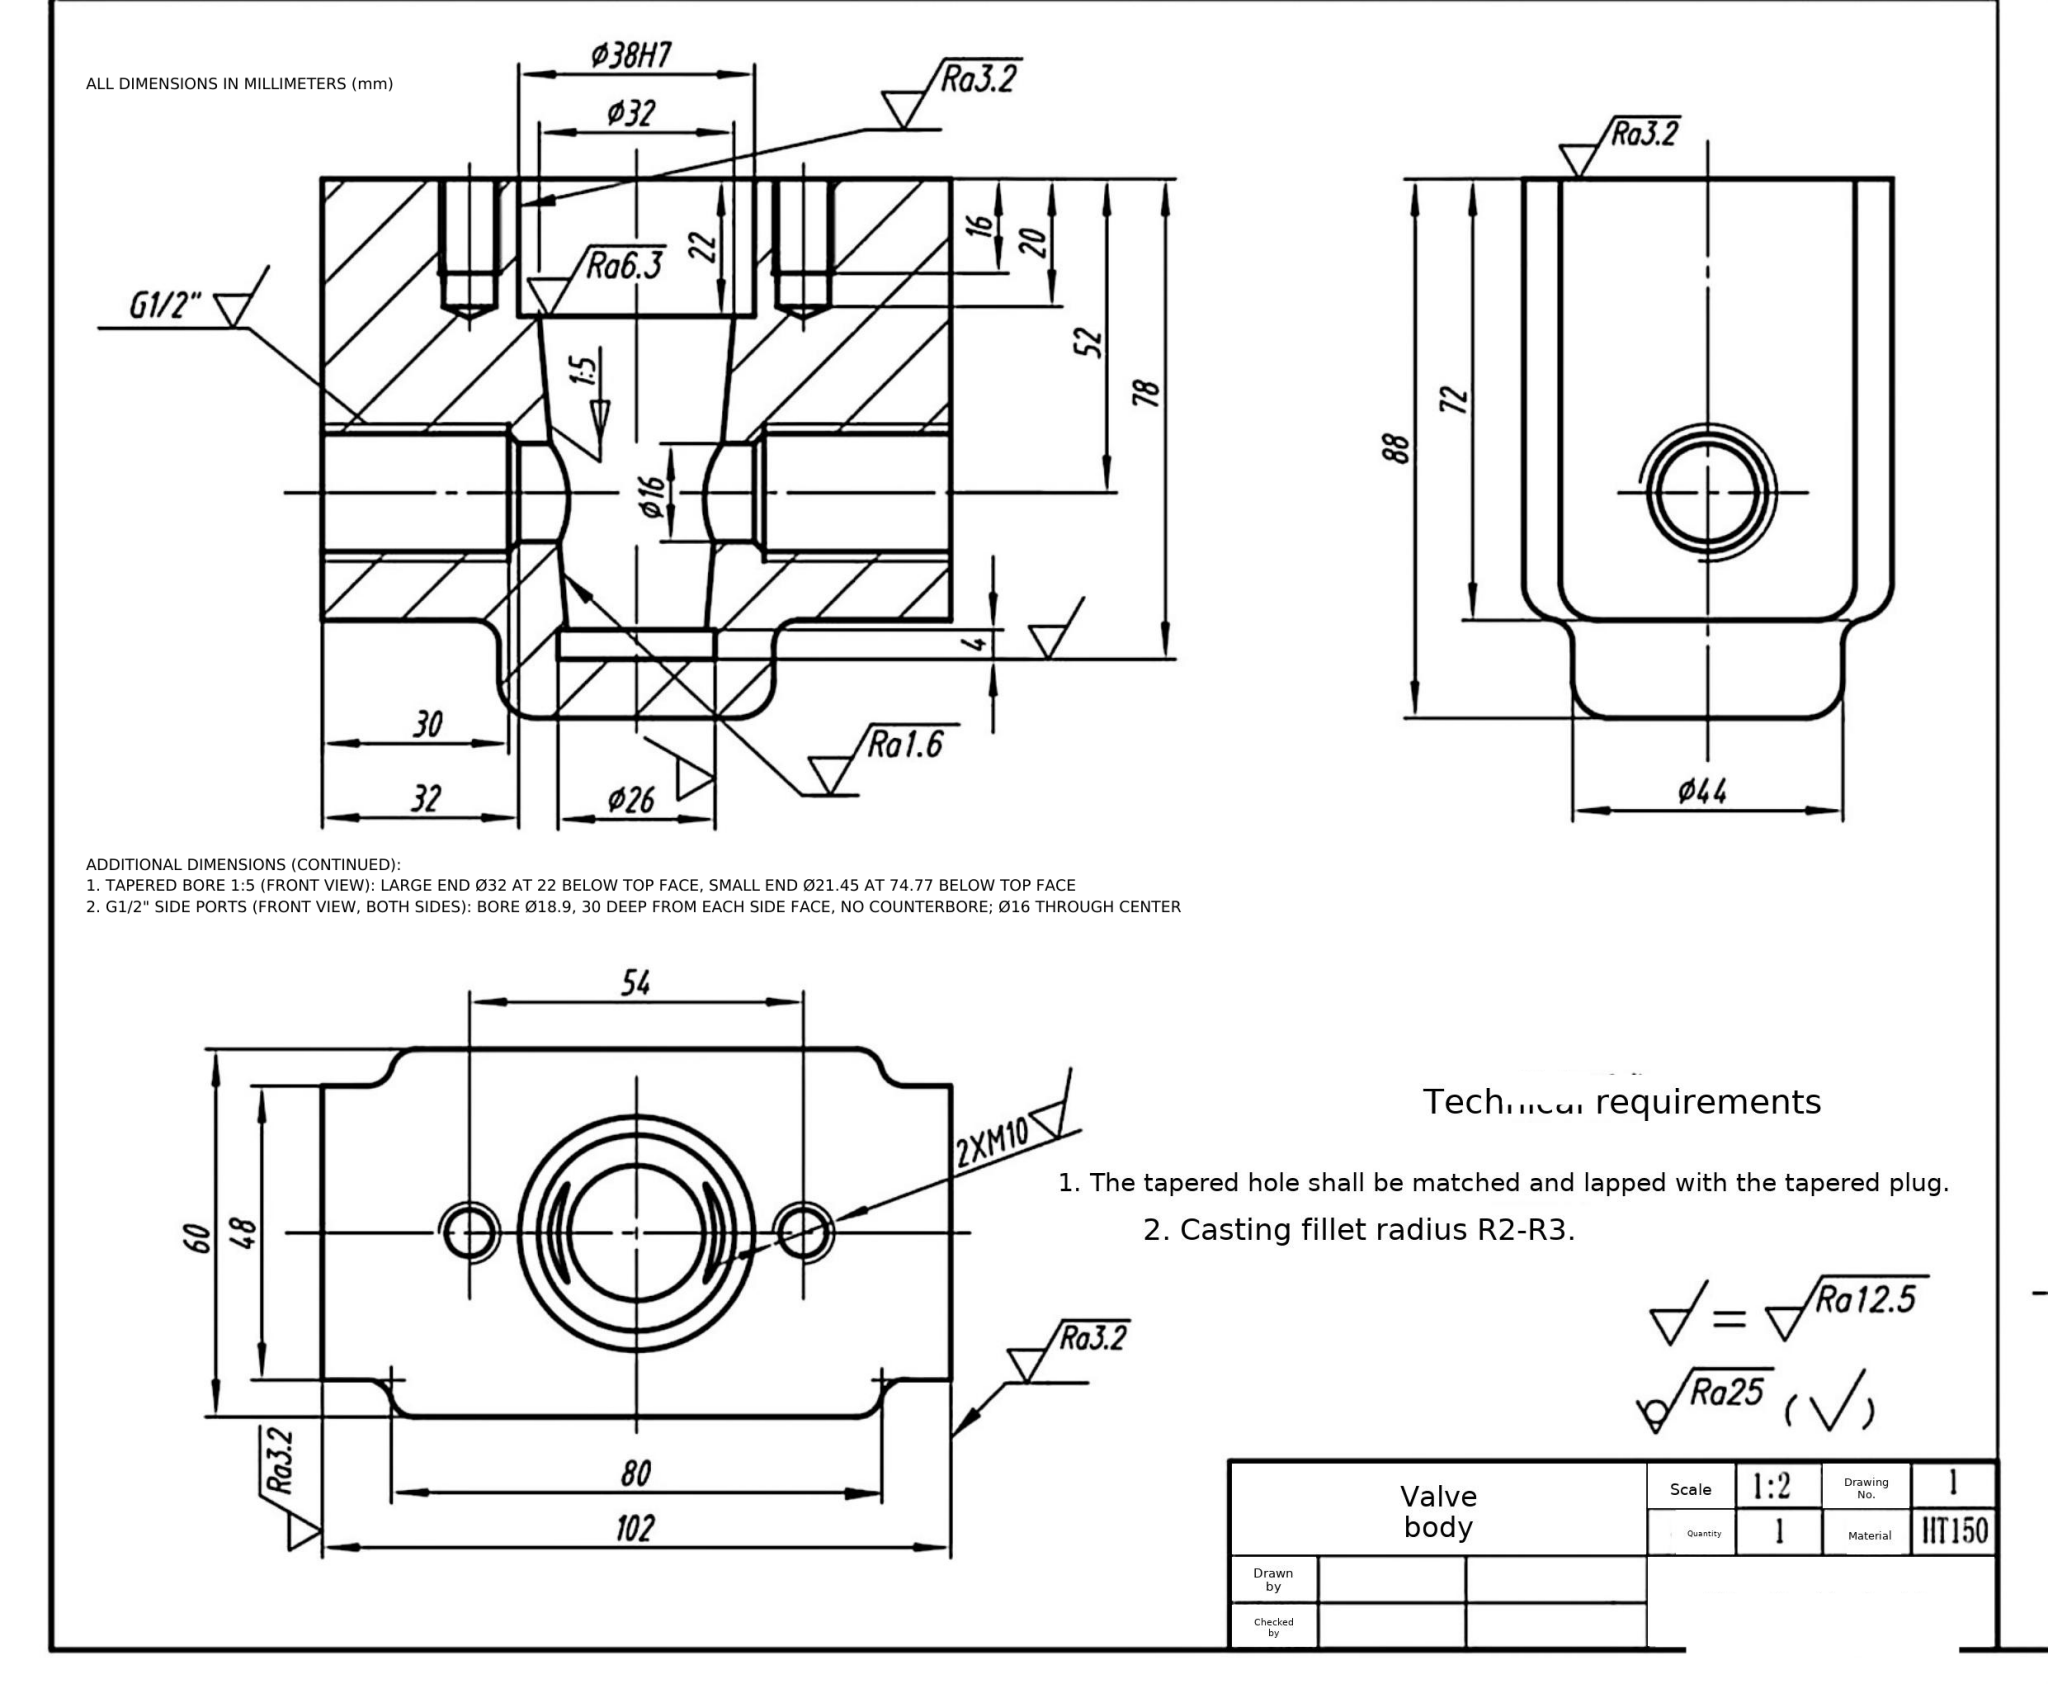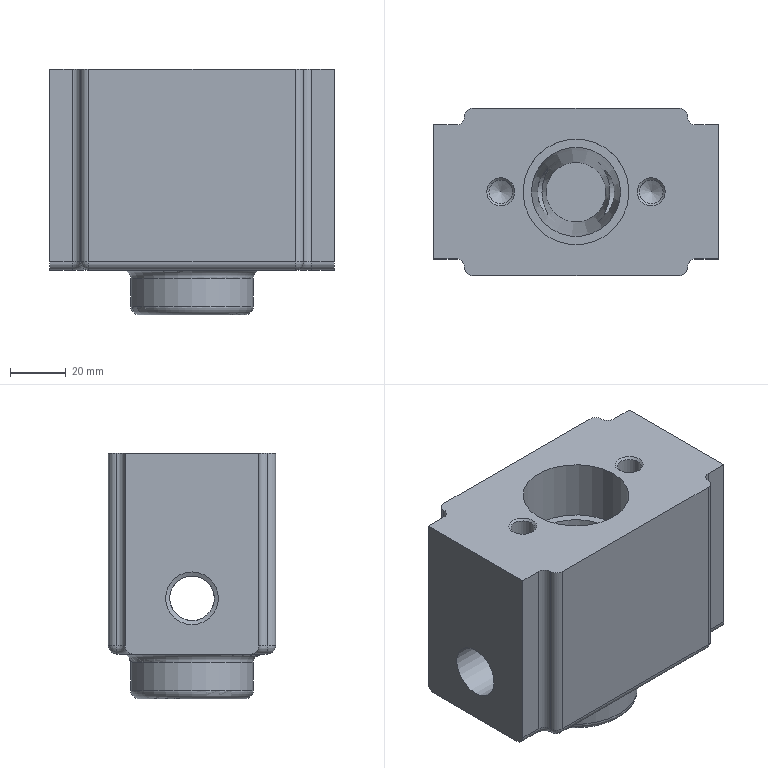Part | NX | mm | 1 solid | 54 faces | box 102 x 60 x 88 mm | volume 365746 mm3 | cylinder 23 | plane 14 | cone 7 | torus 6 | sphere 4 | commonest cylinder face diameters 6 x14 8.5 x2 16 x2 18.9 x2 44 x1 26 x1 38 x1